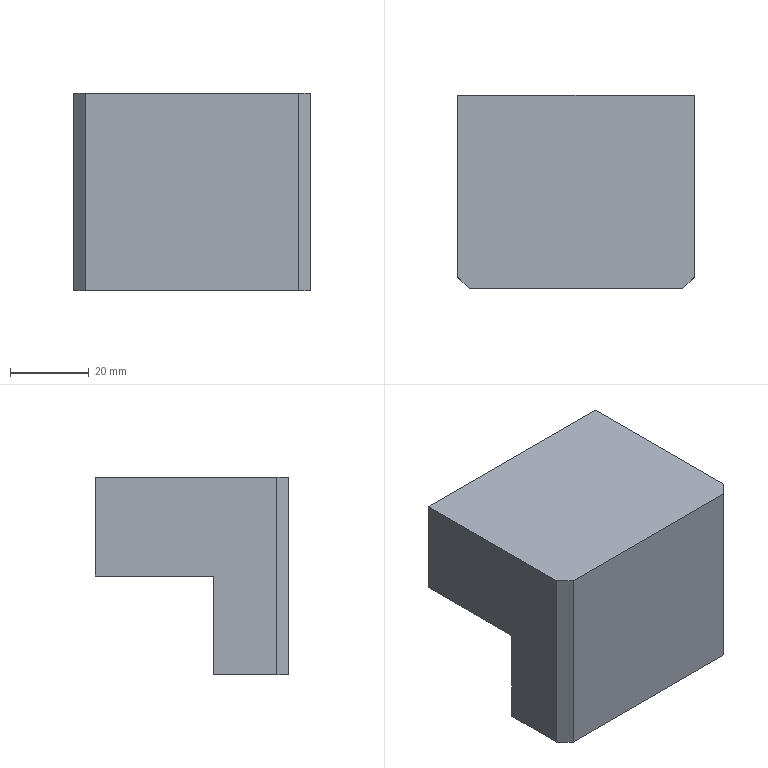Component | SolidWorks | Part51-1 | 1 solid | 10 faces | box 60 x 49 x 50 mm | volume 101550 mm3 | plane 10
build123d program:
from build123d import *

# Parameters (mm, degrees)
BOSS_EXTRUDE1_DEPTH = 30
CHAMFER1_SIZE       = 3


with BuildPart() as part:
    # Sketch1 → Boss-Extrude1 (new, symmetric)
    with BuildSketch(Plane(origin=(0, 0, 0), x_dir=(1, 0, 0), z_dir=(0, 1, 0))):
        Polygon((-49, 0), (0, 0), (0, 50), (-19, 50), (-19, 25), (-49, 25), align=None)
    extrude(amount=BOSS_EXTRUDE1_DEPTH, both=True)

    # Chamfer1
    chamfer1_edges = [part.edges().sort_by_distance(p)[0] for p in [
        (0, 30, -25),
        (0, -30, -25),
    ]]
    chamfer(chamfer1_edges, length=CHAMFER1_SIZE)


solid = part.part

# Placed as in the assembly
solid = solid.moved(Location((-87.007, 369, -360), (0, 0, -90)))
STEP:
#1=COLOUR_RGB('',0.7922,0.8196,0.9333);
#2=FILL_AREA_STYLE_COLOUR('',#1);
#3=FILL_AREA_STYLE('',(#2));
#4=SURFACE_STYLE_FILL_AREA(#3);
#5=SURFACE_SIDE_STYLE('',(#4));
#6=SURFACE_STYLE_USAGE(.BOTH.,#5);
#7=PRESENTATION_STYLE_ASSIGNMENT((#6));
#8=CARTESIAN_POINT('',(-4.607,16.457,-15.157));
#9=VERTEX_POINT('',#8);
#10=CARTESIAN_POINT('',(-4.607,16.457,-14.173));
#11=VERTEX_POINT('',#10);
#12=CARTESIAN_POINT('',(-4.607,16.457,-15.157));
#13=DIRECTION('',(0.,0.,1.));
#14=VECTOR('',#13,39.37);
#15=LINE('',#12,#14);
#16=EDGE_CURVE('',#9,#11,#15,.T.);
#17=ORIENTED_EDGE('',*,*,#16,.T.);
#18=CARTESIAN_POINT('',(-2.244,16.457,-14.173));
#19=VERTEX_POINT('',#18);
#20=CARTESIAN_POINT('',(-2.244,16.457,-14.173));
#21=DIRECTION('',(-1.,0.,0.));
#22=VECTOR('',#21,39.37);
#23=LINE('',#20,#22);
#24=EDGE_CURVE('',#19,#11,#23,.T.);
#25=ORIENTED_EDGE('',*,*,#24,.F.);
#26=CARTESIAN_POINT('',(-2.244,16.457,-15.157));
#27=VERTEX_POINT('',#26);
#28=CARTESIAN_POINT('',(-2.244,16.457,-15.157));
#29=DIRECTION('',(0.,0.,1.));
#30=VECTOR('',#29,39.37);
#31=LINE('',#28,#30);
#32=EDGE_CURVE('',#27,#19,#31,.T.);
#33=ORIENTED_EDGE('',*,*,#32,.F.);
#34=CARTESIAN_POINT('',(-2.244,16.457,-15.157));
#35=DIRECTION('',(-1.,0.,0.));
#36=VECTOR('',#35,39.37);
#37=LINE('',#34,#36);
#38=EDGE_CURVE('',#27,#9,#37,.T.);
#39=ORIENTED_EDGE('',*,*,#38,.T.);
#40=EDGE_LOOP('',(#17,#25,#33,#39));
#41=FACE_OUTER_BOUND('',#40,.T.);
#42=CARTESIAN_POINT('',(-2.244,16.457,-15.157));
#43=DIRECTION('',(0.,-1.,0.));
#44=DIRECTION('',(0.,0.,-1.));
#45=AXIS2_PLACEMENT_3D('',#42,#43,#44);
#46=PLANE('',#45);
#47=ADVANCED_FACE('',(#41),#46,.F.);
#48=CARTESIAN_POINT('',(-2.362,14.528,-14.173));
#49=VERTEX_POINT('',#48);
#50=CARTESIAN_POINT('',(-4.488,14.528,-14.173));
#51=VERTEX_POINT('',#50);
#52=CARTESIAN_POINT('',(-2.244,14.528,-14.173));
#53=DIRECTION('',(-1.,0.,0.));
#54=VECTOR('',#53,39.37);
#55=LINE('',#52,#54);
#56=EDGE_CURVE('',#49,#51,#55,.T.);
#57=ORIENTED_EDGE('',*,*,#56,.F.);
#58=CARTESIAN_POINT('',(-2.244,14.646,-14.173));
#59=VERTEX_POINT('',#58);
#60=CARTESIAN_POINT('',(-2.244,14.646,-14.173));
#61=DIRECTION('',(0.7071,0.7071,0.));
#62=VECTOR('',#61,39.37);
#63=LINE('',#60,#62);
#64=EDGE_CURVE('',#49,#59,#63,.T.);
#65=ORIENTED_EDGE('',*,*,#64,.T.);
#66=CARTESIAN_POINT('',(-2.244,16.457,-14.173));
#67=DIRECTION('',(0.,-1.,0.));
#68=VECTOR('',#67,39.37);
#69=LINE('',#66,#68);
#70=EDGE_CURVE('',#19,#59,#69,.T.);
#71=ORIENTED_EDGE('',*,*,#70,.F.);
#72=ORIENTED_EDGE('',*,*,#24,.T.);
#73=CARTESIAN_POINT('',(-4.607,14.646,-14.173));
#74=VERTEX_POINT('',#73);
#75=CARTESIAN_POINT('',(-4.607,16.457,-14.173));
#76=DIRECTION('',(0.,-1.,0.));
#77=VECTOR('',#76,39.37);
#78=LINE('',#75,#77);
#79=EDGE_CURVE('',#11,#74,#78,.T.);
#80=ORIENTED_EDGE('',*,*,#79,.T.);
#81=CARTESIAN_POINT('',(-4.488,14.528,-14.173));
#82=DIRECTION('',(0.7071,-0.7071,0.));
#83=VECTOR('',#82,39.37);
#84=LINE('',#81,#83);
#85=EDGE_CURVE('',#74,#51,#84,.T.);
#86=ORIENTED_EDGE('',*,*,#85,.T.);
#87=EDGE_LOOP('',(#57,#65,#71,#72,#80,#86));
#88=FACE_OUTER_BOUND('',#87,.T.);
#89=CARTESIAN_POINT('',(-2.244,16.457,-14.173));
#90=DIRECTION('',(0.,0.,-1.));
#91=DIRECTION('',(0.,1.,0.));
#92=AXIS2_PLACEMENT_3D('',#89,#90,#91);
#93=PLANE('',#92);
#94=ADVANCED_FACE('',(#88),#93,.F.);
#95=CARTESIAN_POINT('',(-2.362,14.528,-16.142));
#96=VERTEX_POINT('',#95);
#97=CARTESIAN_POINT('',(-4.488,14.528,-16.142));
#98=VERTEX_POINT('',#97);
#99=CARTESIAN_POINT('',(-2.244,14.528,-16.142));
#100=DIRECTION('',(-1.,0.,0.));
#101=VECTOR('',#100,39.37);
#102=LINE('',#99,#101);
#103=EDGE_CURVE('',#96,#98,#102,.T.);
#104=ORIENTED_EDGE('',*,*,#103,.F.);
#105=CARTESIAN_POINT('',(-2.362,14.528,-14.173));
#106=DIRECTION('',(0.,0.,1.));
#107=VECTOR('',#106,39.37);
#108=LINE('',#105,#107);
#109=EDGE_CURVE('',#96,#49,#108,.T.);
#110=ORIENTED_EDGE('',*,*,#109,.T.);
#111=ORIENTED_EDGE('',*,*,#56,.T.);
#112=CARTESIAN_POINT('',(-4.488,14.528,-14.173));
#113=DIRECTION('',(0.,0.,-1.));
#114=VECTOR('',#113,39.37);
#115=LINE('',#112,#114);
#116=EDGE_CURVE('',#51,#98,#115,.T.);
#117=ORIENTED_EDGE('',*,*,#116,.T.);
#118=EDGE_LOOP('',(#104,#110,#111,#117));
#119=FACE_OUTER_BOUND('',#118,.T.);
#120=CARTESIAN_POINT('',(-2.244,14.528,-14.173));
#121=DIRECTION('',(0.,1.,0.));
#122=DIRECTION('',(0.,0.,1.));
#123=AXIS2_PLACEMENT_3D('',#120,#121,#122);
#124=PLANE('',#123);
#125=ADVANCED_FACE('',(#119),#124,.F.);
#126=CARTESIAN_POINT('',(-2.244,14.646,-16.142));
#127=VERTEX_POINT('',#126);
#128=CARTESIAN_POINT('',(-2.244,15.276,-16.142));
#129=VERTEX_POINT('',#128);
#130=CARTESIAN_POINT('',(-2.244,14.528,-16.142));
#131=DIRECTION('',(0.,1.,0.));
#132=VECTOR('',#131,39.37);
#133=LINE('',#130,#132);
#134=EDGE_CURVE('',#127,#129,#133,.T.);
#135=ORIENTED_EDGE('',*,*,#134,.F.);
#136=CARTESIAN_POINT('',(-2.244,14.646,-16.142));
#137=DIRECTION('',(-0.7071,-0.7071,0.));
#138=VECTOR('',#137,39.37);
#139=LINE('',#136,#138);
#140=EDGE_CURVE('',#127,#96,#139,.T.);
#141=ORIENTED_EDGE('',*,*,#140,.T.);
#142=ORIENTED_EDGE('',*,*,#103,.T.);
#143=CARTESIAN_POINT('',(-4.607,14.646,-16.142));
#144=VERTEX_POINT('',#143);
#145=CARTESIAN_POINT('',(-4.488,14.528,-16.142));
#146=DIRECTION('',(-0.7071,0.7071,0.));
#147=VECTOR('',#146,39.37);
#148=LINE('',#145,#147);
#149=EDGE_CURVE('',#98,#144,#148,.T.);
#150=ORIENTED_EDGE('',*,*,#149,.T.);
#151=CARTESIAN_POINT('',(-4.607,15.276,-16.142));
#152=VERTEX_POINT('',#151);
#153=CARTESIAN_POINT('',(-4.607,14.528,-16.142));
#154=DIRECTION('',(0.,1.,0.));
#155=VECTOR('',#154,39.37);
#156=LINE('',#153,#155);
#157=EDGE_CURVE('',#144,#152,#156,.T.);
#158=ORIENTED_EDGE('',*,*,#157,.T.);
#159=CARTESIAN_POINT('',(-2.244,15.276,-16.142));
#160=DIRECTION('',(-1.,0.,0.));
#161=VECTOR('',#160,39.37);
#162=LINE('',#159,#161);
#163=EDGE_CURVE('',#129,#152,#162,.T.);
#164=ORIENTED_EDGE('',*,*,#163,.F.);
#165=EDGE_LOOP('',(#135,#141,#142,#150,#158,#164));
#166=FACE_OUTER_BOUND('',#165,.T.);
#167=CARTESIAN_POINT('',(-2.244,14.528,-16.142));
#168=DIRECTION('',(0.,0.,1.));
#169=DIRECTION('',(0.,-1.,0.));
#170=AXIS2_PLACEMENT_3D('',#167,#168,#169);
#171=PLANE('',#170);
#172=ADVANCED_FACE('',(#166),#171,.F.);
#173=CARTESIAN_POINT('',(-4.607,15.276,-15.157));
#174=VERTEX_POINT('',#173);
#175=CARTESIAN_POINT('',(-4.607,15.276,-16.142));
#176=DIRECTION('',(0.,-0.,1.));
#177=VECTOR('',#176,39.37);
#178=LINE('',#175,#177);
#179=EDGE_CURVE('',#152,#174,#178,.T.);
#180=ORIENTED_EDGE('',*,*,#179,.T.);
#181=CARTESIAN_POINT('',(-2.244,15.276,-15.157));
#182=VERTEX_POINT('',#181);
#183=CARTESIAN_POINT('',(-2.244,15.276,-15.157));
#184=DIRECTION('',(-1.,0.,0.));
#185=VECTOR('',#184,39.37);
#186=LINE('',#183,#185);
#187=EDGE_CURVE('',#182,#174,#186,.T.);
#188=ORIENTED_EDGE('',*,*,#187,.F.);
#189=CARTESIAN_POINT('',(-2.244,15.276,-16.142));
#190=DIRECTION('',(0.,-0.,1.));
#191=VECTOR('',#190,39.37);
#192=LINE('',#189,#191);
#193=EDGE_CURVE('',#129,#182,#192,.T.);
#194=ORIENTED_EDGE('',*,*,#193,.F.);
#195=ORIENTED_EDGE('',*,*,#163,.T.);
#196=EDGE_LOOP('',(#180,#188,#194,#195));
#197=FACE_OUTER_BOUND('',#196,.T.);
#198=CARTESIAN_POINT('',(-2.244,15.276,-16.142));
#199=DIRECTION('',(0.,-1.,-0.));
#200=DIRECTION('',(0.,0.,-1.));
#201=AXIS2_PLACEMENT_3D('',#198,#199,#200);
#202=PLANE('',#201);
#203=ADVANCED_FACE('',(#197),#202,.F.);
#204=CARTESIAN_POINT('',(-4.607,15.276,-15.157));
#205=DIRECTION('',(0.,1.,0.));
#206=VECTOR('',#205,39.37);
#207=LINE('',#204,#206);
#208=EDGE_CURVE('',#174,#9,#207,.T.);
#209=ORIENTED_EDGE('',*,*,#208,.T.);
#210=ORIENTED_EDGE('',*,*,#38,.F.);
#211=CARTESIAN_POINT('',(-2.244,15.276,-15.157));
#212=DIRECTION('',(0.,1.,0.));
#213=VECTOR('',#212,39.37);
#214=LINE('',#211,#213);
#215=EDGE_CURVE('',#182,#27,#214,.T.);
#216=ORIENTED_EDGE('',*,*,#215,.F.);
#217=ORIENTED_EDGE('',*,*,#187,.T.);
#218=EDGE_LOOP('',(#209,#210,#216,#217));
#219=FACE_OUTER_BOUND('',#218,.T.);
#220=CARTESIAN_POINT('',(-2.244,15.276,-15.157));
#221=DIRECTION('',(0.,0.,1.));
#222=DIRECTION('',(0.,-1.,0.));
#223=AXIS2_PLACEMENT_3D('',#220,#221,#222);
#224=PLANE('',#223);
#225=ADVANCED_FACE('',(#219),#224,.F.);
#226=ORIENTED_EDGE('',*,*,#70,.T.);
#227=CARTESIAN_POINT('',(-2.244,14.646,-16.142));
#228=DIRECTION('',(0.,0.,-1.));
#229=VECTOR('',#228,39.37);
#230=LINE('',#227,#229);
#231=EDGE_CURVE('',#59,#127,#230,.T.);
#232=ORIENTED_EDGE('',*,*,#231,.T.);
#233=ORIENTED_EDGE('',*,*,#134,.T.);
#234=ORIENTED_EDGE('',*,*,#193,.T.);
#235=ORIENTED_EDGE('',*,*,#215,.T.);
#236=ORIENTED_EDGE('',*,*,#32,.T.);
#237=EDGE_LOOP('',(#226,#232,#233,#234,#235,#236));
#238=FACE_OUTER_BOUND('',#237,.T.);
#239=CARTESIAN_POINT('',(-2.244,14.528,-14.173));
#240=DIRECTION('',(1.,0.,0.));
#241=DIRECTION('',(0.,0.,1.));
#242=AXIS2_PLACEMENT_3D('',#239,#240,#241);
#243=PLANE('',#242);
#244=ADVANCED_FACE('',(#238),#243,.T.);
#245=ORIENTED_EDGE('',*,*,#157,.F.);
#246=CARTESIAN_POINT('',(-4.607,14.646,-14.173));
#247=DIRECTION('',(0.,0.,1.));
#248=VECTOR('',#247,39.37);
#249=LINE('',#246,#248);
#250=EDGE_CURVE('',#144,#74,#249,.T.);
#251=ORIENTED_EDGE('',*,*,#250,.T.);
#252=ORIENTED_EDGE('',*,*,#79,.F.);
#253=ORIENTED_EDGE('',*,*,#16,.F.);
#254=ORIENTED_EDGE('',*,*,#208,.F.);
#255=ORIENTED_EDGE('',*,*,#179,.F.);
#256=EDGE_LOOP('',(#245,#251,#252,#253,#254,#255));
#257=FACE_OUTER_BOUND('',#256,.T.);
#258=CARTESIAN_POINT('',(-4.607,14.528,-14.173));
#259=DIRECTION('',(1.,0.,0.));
#260=DIRECTION('',(0.,0.,1.));
#261=AXIS2_PLACEMENT_3D('',#258,#259,#260);
#262=PLANE('',#261);
#263=ADVANCED_FACE('',(#257),#262,.F.);
#264=ORIENTED_EDGE('',*,*,#64,.F.);
#265=ORIENTED_EDGE('',*,*,#109,.F.);
#266=ORIENTED_EDGE('',*,*,#140,.F.);
#267=ORIENTED_EDGE('',*,*,#231,.F.);
#268=EDGE_LOOP('',(#264,#265,#266,#267));
#269=FACE_OUTER_BOUND('',#268,.T.);
#270=CARTESIAN_POINT('',(-2.244,14.646,-14.173));
#271=DIRECTION('',(0.7071,-0.7071,0.));
#272=DIRECTION('',(0.,0.,1.));
#273=AXIS2_PLACEMENT_3D('',#270,#271,#272);
#274=PLANE('',#273);
#275=ADVANCED_FACE('',(#269),#274,.T.);
#276=ORIENTED_EDGE('',*,*,#85,.F.);
#277=ORIENTED_EDGE('',*,*,#250,.F.);
#278=ORIENTED_EDGE('',*,*,#149,.F.);
#279=ORIENTED_EDGE('',*,*,#116,.F.);
#280=EDGE_LOOP('',(#276,#277,#278,#279));
#281=FACE_OUTER_BOUND('',#280,.T.);
#282=CARTESIAN_POINT('',(-4.488,14.528,-14.173));
#283=DIRECTION('',(0.7071,0.7071,0.));
#284=DIRECTION('',(0.,0.,-1.));
#285=AXIS2_PLACEMENT_3D('',#282,#283,#284);
#286=PLANE('',#285);
#287=ADVANCED_FACE('',(#281),#286,.F.);
#288=CLOSED_SHELL('',(#47,#94,#125,#172,#203,#225,#244,#263,#275,#287));
#289=MANIFOLD_SOLID_BREP('',#288);
#290=STYLED_ITEM('',(#7),#289);
#291=PRESENTATION_LAYER_ASSIGNMENT('','',(#290));
#292=CARTESIAN_POINT('',(0.,0.,0.));
#293=DIRECTION('',(0.,0.,1.));
#294=DIRECTION('',(1.,0.,0.));
#295=AXIS2_PLACEMENT_3D('',#292,#293,#294);
#296=(LENGTH_UNIT()NAMED_UNIT(*)SI_UNIT($,.METRE.));
#297=LENGTH_MEASURE_WITH_UNIT(LENGTH_MEASURE(0.0254),#296);
#298=DIMENSIONAL_EXPONENTS(1.,0.,0.,0.,0.,0.,0.);
#299=(CONVERSION_BASED_UNIT('',#297)LENGTH_UNIT()NAMED_UNIT(#298));
#300=UNCERTAINTY_MEASURE_WITH_UNIT(LENGTH_MEASURE(0.00001),#299,'','');
#301=(NAMED_UNIT(*)PLANE_ANGLE_UNIT()SI_UNIT($,.RADIAN.));
#302=(NAMED_UNIT(*)SI_UNIT($,.STERADIAN.)SOLID_ANGLE_UNIT());
#303=(GEOMETRIC_REPRESENTATION_CONTEXT(3)GLOBAL_UNCERTAINTY_ASSIGNED_CONTEXT((#300))GLOBAL_UNIT_ASSIGNED_CONTEXT((#299,#301,#302))REPRESENTATION_CONTEXT('',''));
#304=ADVANCED_BREP_SHAPE_REPRESENTATION('',(#289,#295),#303);
#305=(LENGTH_UNIT()NAMED_UNIT(*)SI_UNIT($,.METRE.));
#306=LENGTH_MEASURE_WITH_UNIT(LENGTH_MEASURE(0.0254),#305);
#307=DIMENSIONAL_EXPONENTS(1.,0.,0.,0.,0.,0.,0.);
#308=(CONVERSION_BASED_UNIT('',#306)LENGTH_UNIT()NAMED_UNIT(#307));
#309=UNCERTAINTY_MEASURE_WITH_UNIT(LENGTH_MEASURE(0.00001),#308,'','');
#310=(NAMED_UNIT(*)PLANE_ANGLE_UNIT()SI_UNIT($,.RADIAN.));
#311=(NAMED_UNIT(*)SI_UNIT($,.STERADIAN.)SOLID_ANGLE_UNIT());
#312=(GEOMETRIC_REPRESENTATION_CONTEXT(3)GLOBAL_UNCERTAINTY_ASSIGNED_CONTEXT((#309))GLOBAL_UNIT_ASSIGNED_CONTEXT((#308,#310,#311))REPRESENTATION_CONTEXT('',''));
#313=MECHANICAL_DESIGN_GEOMETRIC_PRESENTATION_REPRESENTATION('',(#290),#312);